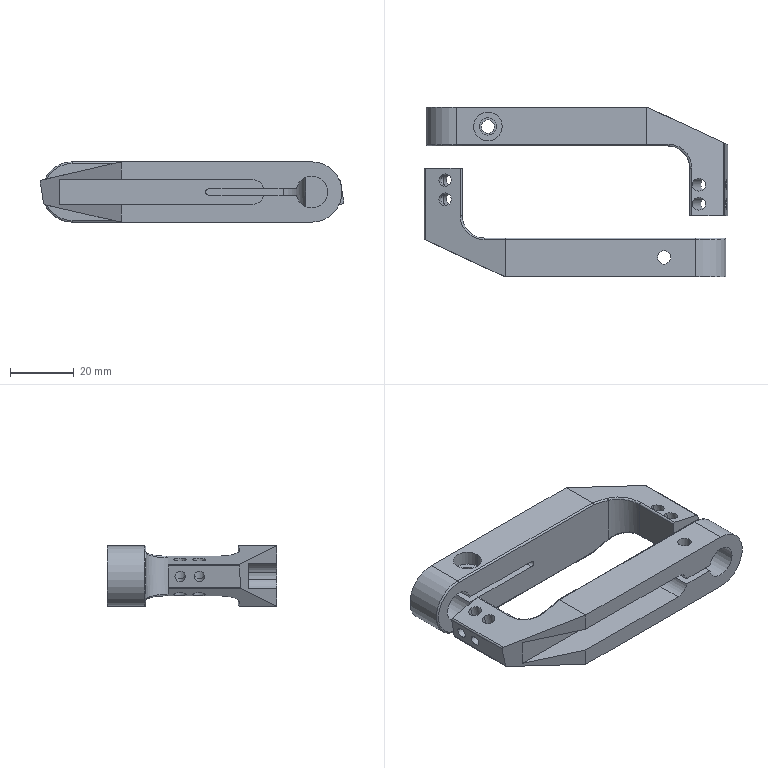CAM job | Mastercam | mm | 1 operations | part box 106.09 x 53.4 x 19
1. Contour (Ramp) | 1 - 6 平铣刀